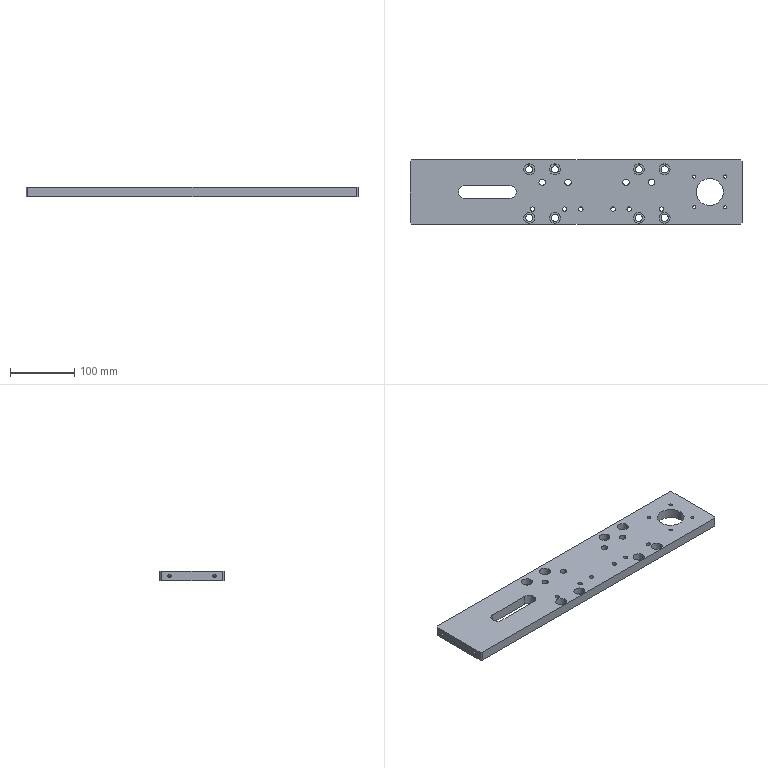Component | SolidWorks | -UpperSlidingSleeveConnectingPlate02-1 | 1 solid | 93 faces | box 515 x 100 x 15 mm | volume 692874 mm3 | cylinder 69 | plane 20 | cone 4 | commonest cylinder face diameters 17 x16 11 x16 5 x12 6.8 x12 10 x8 20 x3 42 x2
build123d program:
from build123d import *

# Parameters (mm, degrees)
SKETCH1_W                                            = 515
SKETCH1_H                                            = 100
BOSS_EXTRUDE1_DEPTH                                  = 7.5
CYLINDRICAL_COUNTERSUNK_HOLE_FOR_M10_HEX_D           = 11
CYLINDRICAL_COUNTERSUNK_HOLE_FOR_M10_HEX_DEPTH       = 22.25
CYLINDRICAL_COUNTERSUNK_HOLE_FOR_M10_HEX_CBORE_D     = 17
CYLINDRICAL_COUNTERSUNK_HOLE_FOR_M10_HEX_CBORE_DEPTH = 11
CYLINDRICAL_COUNTERSUNK_HOLE_FOR_M10_HEX_TIP         = 3.305
M8_TAPPED_HOLE1_D                                    = 6.8
M8_TAPPED_HOLE1_DEPTH                                = 22.25
M8_TAPPED_HOLE1_TIP                                  = 2.043
SKETCH8_R                                            = 21
CUT_EXTRUDE1_DEPTH                                   = 15
CIRPATTERN1_COUNT                                    = 4
CUT_EXTRUDE2_DEPTH                                   = 15
M6_TAPPED_HOLE1_D                                    = 5
M6_TAPPED_HOLE1_DEPTH                                = 17
M6_TAPPED_HOLE1_TIP                                  = 1.502
M10_TAPPED_HOLE1_D                                   = 10
CHAMFER1_SIZE                                        = 3
M10_TAPPED_HOLE2_D                                   = 10


with BuildPart() as part:
    # Sketch1 → Boss-Extrude1 (new, symmetric)
    with BuildSketch(Plane.XY):
        Rectangle(SKETCH1_W, SKETCH1_H)
    extrude(amount=BOSS_EXTRUDE1_DEPTH, both=True)

    # Cylindrical Countersunk Hole for M10 Hex
    with Locations(Plane.XY.offset(7.5)):
        with Locations((97.5, 35), (97.5, -40), (137.5, 35), (137.5, -40), (-32.5, -40), (-32.5, 35), (-72.5, 35), (-72.5, -40)):
            CounterBoreHole(CYLINDRICAL_COUNTERSUNK_HOLE_FOR_M10_HEX_D / 2, CYLINDRICAL_COUNTERSUNK_HOLE_FOR_M10_HEX_CBORE_D / 2, CYLINDRICAL_COUNTERSUNK_HOLE_FOR_M10_HEX_CBORE_DEPTH, depth=CYLINDRICAL_COUNTERSUNK_HOLE_FOR_M10_HEX_DEPTH)
            with Locations((0, 0, -(CYLINDRICAL_COUNTERSUNK_HOLE_FOR_M10_HEX_DEPTH + CYLINDRICAL_COUNTERSUNK_HOLE_FOR_M10_HEX_TIP / 2))):  # 118° drill point
                Cone(0, CYLINDRICAL_COUNTERSUNK_HOLE_FOR_M10_HEX_D / 2, CYLINDRICAL_COUNTERSUNK_HOLE_FOR_M10_HEX_TIP, mode=Mode.SUBTRACT)

    # M8 Tapped Hole1
    with Locations(Plane.XY.offset(7.5)):
        with Locations((132.5, -26.5), (82.5, -26.5), (57.5, -26.5), (7.5, -26.5), (-17.5, -26.5), (-67.5, -26.5)):
            Hole(M8_TAPPED_HOLE1_D / 2, depth=M8_TAPPED_HOLE1_DEPTH)
            with Locations((0, 0, -(M8_TAPPED_HOLE1_DEPTH + M8_TAPPED_HOLE1_TIP / 2))):  # 118° drill point
                Cone(0, M8_TAPPED_HOLE1_D / 2, M8_TAPPED_HOLE1_TIP, mode=Mode.SUBTRACT)

    # Sketch8 → Cut-Extrude1 (cut)
    with BuildSketch(Plane.XY.offset(7.5)):
        with Locations((207.5, 0)):
            Circle(SKETCH8_R)
    extrude(amount=-CUT_EXTRUDE1_DEPTH, mode=Mode.SUBTRACT)

    # Sketch9 → M6 Tapped Hole2 (revolve, cut)
    with BuildSketch(Plane(origin=(183.635, 23.865, 7.5), x_dir=(0, -1, 0), z_dir=(1, 0, 0))):
        Polygon((0, 0), (0, 18.502), (2.5, 17), (2.5, 0), align=None)
    m6_tapped_hole2 = revolve(axis=Axis((183.635, 23.865, 13.85), (0, 0, -1)), mode=Mode.SUBTRACT)

    # CirPattern1: M6 Tapped Hole2 ×4 about axis
    cirpattern1_axis = Axis((207.5, 0, 0), (0, 0, 1))
    for i in range(1, CIRPATTERN1_COUNT):
        add(m6_tapped_hole2.rotate(cirpattern1_axis, i * 360 / CIRPATTERN1_COUNT), mode=Mode.SUBTRACT)

    # Sketch11 → Cut-Extrude2 (cut)
    with BuildSketch(Plane.XY.offset(7.5)):
        with BuildLine():
            Line((-172.5, 10), (-102.5, 10))
            ThreePointArc((-102.5, 10), (-92.5, 0), (-102.5, -10))
            Line((-102.5, -10), (-172.5, -10))
            ThreePointArc((-172.5, -10), (-182.5, 0), (-172.5, 10))
        make_face()
    extrude(amount=-CUT_EXTRUDE2_DEPTH, mode=Mode.SUBTRACT)

    # M6 Tapped Hole1
    with Locations(Plane.ZY.offset(257.5)):
        with Locations((0, 35), (0, -35)):
            Hole(M6_TAPPED_HOLE1_D / 2, depth=M6_TAPPED_HOLE1_DEPTH)
            with Locations((0, 0, -(M6_TAPPED_HOLE1_DEPTH + M6_TAPPED_HOLE1_TIP / 2))):  # 118° drill point
                Cone(0, M6_TAPPED_HOLE1_D / 2, M6_TAPPED_HOLE1_TIP, mode=Mode.SUBTRACT)

    # M10 Tapped Hole1 (through all)
    with Locations(Plane(origin=(0, 0, -7.5), x_dir=(1, 0, 0), z_dir=(0, 0, -1))):
        with Locations((-52.5, -15), (117.5, -15)):
            Hole(M10_TAPPED_HOLE1_D / 2)

    # Chamfer1
    chamfer1_edges = [part.edges().sort_by_distance(p)[0] for p in [
        (-257.5, 50, 0),
        (257.5, 50, 0),
        (257.5, -50, 0),
        (-257.5, -50, 0),
    ]]
    chamfer(chamfer1_edges, length=CHAMFER1_SIZE)

    # M10 Tapped Hole2 (through all)
    with Locations(Plane(origin=(0, 0, -7.5), x_dir=(-1, 0, 0), z_dir=(0, 0, -1))):
        with Locations((-77.5, 15), (12.5, 15)):
            Hole(M10_TAPPED_HOLE2_D / 2)


solid = part.part

# Placed as in the assembly
solid = solid.moved(Location((-2.5, 1239.5, -2.5), (0, 0, 0)))